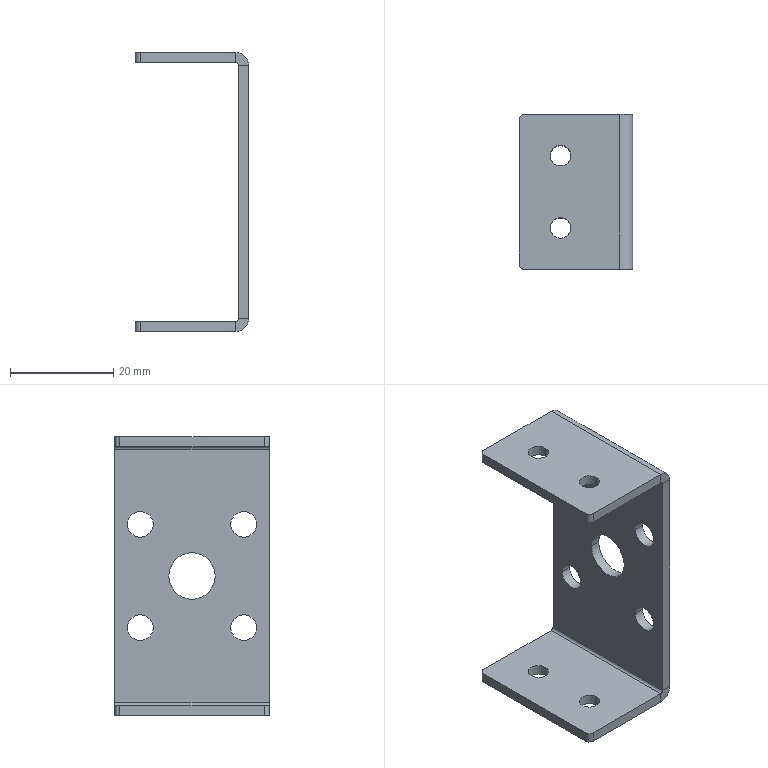Component | SolidWorks | InnerBagClampingCylinderFixingPlate-1 | 1 solid | 44 faces | volume 5176 mm3 | cylinder 26 | plane 18 | commonest cylinder face diameters 5 x10 4 x8 2 x4 9 x2 1 x2